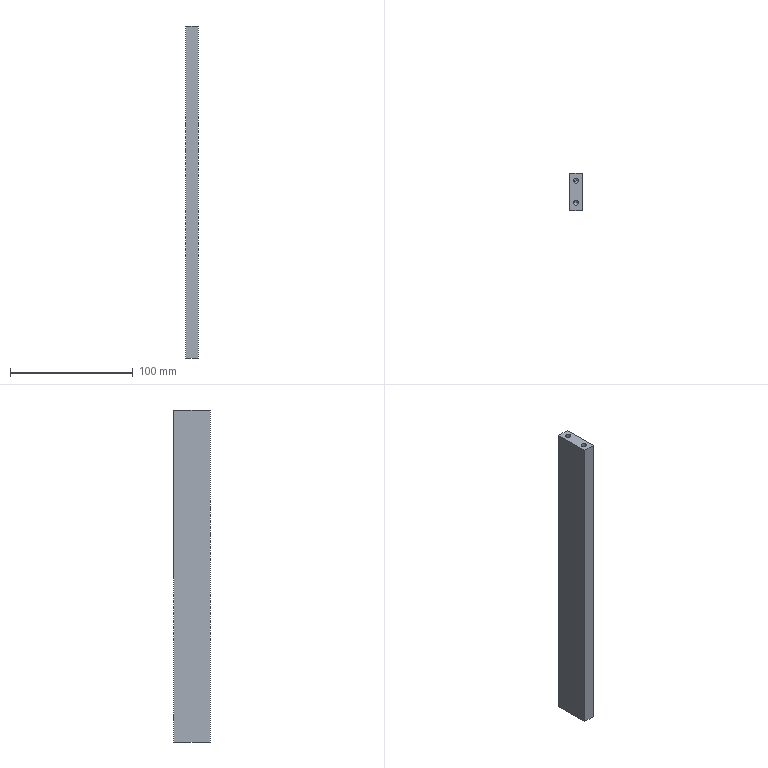Component | SolidWorks | LD101-02--Q1033-Q1-2-1 | 1 solid | 34 faces | box 10 x 30 x 270 mm | volume 79735 mm3 | cylinder 14 | cone 14 | plane 6 | commonest cylinder face diameters 4.2 x8 3.3 x6 | material AL6061
build123d program:
from build123d import *

# Parameters (mm, degrees)
SKETCH1_W                  = 270
SKETCH1_H                  = 30
BOSS_EXTRUDE1_DEPTH        = 5
M5_TAPPED_HOLE1_AT_2_COUNT = 2
M5_TAPPED_HOLE1_AT_2_PITCH = 18
M4_TAPPED_HOLE2_D          = 3.3
M4_TAPPED_HOLE2_DEPTH      = 13.5
M4_TAPPED_HOLE2_TIP        = 0.9914


with BuildPart() as part:
    # Sketch1 → Boss-Extrude1 (new, symmetric)
    with BuildSketch(Plane.XY):
        Rectangle(SKETCH1_W, SKETCH1_H)
    extrude(amount=BOSS_EXTRUDE1_DEPTH, both=True)

    # Sketch2 → M5 Tapped Hole1 (revolve, cut)
    with BuildSketch(Plane(origin=(135, -9, 0), x_dir=(0, 0, -1), z_dir=(0, 1, 0))):
        Polygon((0, 0), (0, 17.262), (2.1, 16), (2.1, 0), align=None)
    m5_tapped_hole1 = revolve(axis=Axis((141.35, -9, 0), (-1, 0, 0)), mode=Mode.SUBTRACT)

    # M5 Tapped Hole1 at 2: M5 Tapped Hole1 ×2
    with Locations(*[(0, i * M5_TAPPED_HOLE1_AT_2_PITCH, 0) for i in range(1, M5_TAPPED_HOLE1_AT_2_COUNT)]):
        add(m5_tapped_hole1, mode=Mode.SUBTRACT)

    # Mirror1: M5 Tapped Hole1 across plane
    add(m5_tapped_hole1.mirror(Plane(origin=(0, 0, 0), x_dir=(0, 0, 1), z_dir=(1, 0, 0))), mode=Mode.SUBTRACT)

    # Mirror1 copy 1 sketch → Mirror1 copy 1 (revolve, cut)
    with BuildSketch(Plane(origin=(-135, 9, 0), x_dir=(0, 0, -1), z_dir=(0, 1, 0))):
        Polygon((0, 0), (0, -17.262), (2.1, -16), (2.1, 0), align=None)
    revolve(axis=Axis((-141.35, 9, 0), (-1, 0, 0)), mode=Mode.SUBTRACT)

    # M4 Tapped Hole2
    with Locations(Plane(origin=(0, 15, 0), x_dir=(1, 0, 0), z_dir=(0, 1, 0))):
        with Locations((-115, 0), (115, 0), (0, 0)):
            Hole(M4_TAPPED_HOLE2_D / 2, depth=M4_TAPPED_HOLE2_DEPTH)
            with Locations((0, 0, -(M4_TAPPED_HOLE2_DEPTH + M4_TAPPED_HOLE2_TIP / 2))):  # 118° drill point
                Cone(0, M4_TAPPED_HOLE2_D / 2, M4_TAPPED_HOLE2_TIP, mode=Mode.SUBTRACT)


solid = part.part

# Placed as in the assembly
solid = solid.moved(Location((-345.29, -171.897, 146.257), (0, 90, 0)))
STEP:
#1=COLOUR_RGB('',0.7922,0.8196,0.9333);
#2=FILL_AREA_STYLE_COLOUR('',#1);
#3=FILL_AREA_STYLE('',(#2));
#4=SURFACE_STYLE_FILL_AREA(#3);
#5=SURFACE_SIDE_STYLE('',(#4));
#6=SURFACE_STYLE_USAGE(.BOTH.,#5);
#7=PRESENTATION_STYLE_ASSIGNMENT((#6));
#8=CARTESIAN_POINT('',(-13.529,-6.709,1.231));
#9=VERTEX_POINT('',#8);
#10=CARTESIAN_POINT('',(-13.659,-6.709,1.231));
#11=VERTEX_POINT('',#10);
#12=CARTESIAN_POINT('',(-13.594,-6.709,1.231));
#13=DIRECTION('',(0.,1.,0.));
#14=DIRECTION('',(-1.,0.,0.));
#15=AXIS2_PLACEMENT_3D('',#12,#13,#14);
#16=CIRCLE('',#15,0.06496);
#17=EDGE_CURVE('',#9,#11,#16,.T.);
#18=ORIENTED_EDGE('',*,*,#17,.F.);
#19=CARTESIAN_POINT('',(-13.529,-6.177,1.231));
#20=VERTEX_POINT('',#19);
#21=CARTESIAN_POINT('',(-13.529,-6.177,1.231));
#22=DIRECTION('',(0.,1.,0.));
#23=VECTOR('',#22,39.37);
#24=LINE('',#21,#23);
#25=EDGE_CURVE('',#9,#20,#24,.T.);
#26=ORIENTED_EDGE('',*,*,#25,.T.);
#27=CARTESIAN_POINT('',(-13.659,-6.177,1.231));
#28=VERTEX_POINT('',#27);
#29=CARTESIAN_POINT('',(-13.594,-6.177,1.231));
#30=DIRECTION('',(0.,1.,0.));
#31=DIRECTION('',(-1.,0.,0.));
#32=AXIS2_PLACEMENT_3D('',#29,#30,#31);
#33=CIRCLE('',#32,0.06496);
#34=EDGE_CURVE('',#20,#28,#33,.T.);
#35=ORIENTED_EDGE('',*,*,#34,.T.);
#36=CARTESIAN_POINT('',(-13.659,-6.177,1.231));
#37=DIRECTION('',(0.,1.,0.));
#38=VECTOR('',#37,39.37);
#39=LINE('',#36,#38);
#40=EDGE_CURVE('',#11,#28,#39,.T.);
#41=ORIENTED_EDGE('',*,*,#40,.F.);
#42=EDGE_LOOP('',(#18,#26,#35,#41));
#43=FACE_OUTER_BOUND('',#42,.T.);
#44=CARTESIAN_POINT('',(-13.594,-6.177,1.231));
#45=DIRECTION('',(0.,1.,0.));
#46=DIRECTION('',(-1.,0.,0.));
#47=AXIS2_PLACEMENT_3D('',#44,#45,#46);
#48=CYLINDRICAL_SURFACE('',#47,0.06496);
#49=ADVANCED_FACE('',(#43),#48,.F.);
#50=CARTESIAN_POINT('',(-13.594,-6.748,1.231));
#51=VERTEX_POINT('',#50);
#52=CARTESIAN_POINT('',(-13.659,-6.709,1.231));
#53=DIRECTION('',(-0.8572,0.515,0.));
#54=VECTOR('',#53,39.37);
#55=LINE('',#52,#54);
#56=EDGE_CURVE('',#51,#11,#55,.T.);
#57=ORIENTED_EDGE('',*,*,#56,.F.);
#58=CARTESIAN_POINT('',(-13.529,-6.709,1.231));
#59=DIRECTION('',(0.8572,0.515,0.));
#60=VECTOR('',#59,39.37);
#61=LINE('',#58,#60);
#62=EDGE_CURVE('',#51,#9,#61,.T.);
#63=ORIENTED_EDGE('',*,*,#62,.T.);
#64=ORIENTED_EDGE('',*,*,#17,.T.);
#65=EDGE_LOOP('',(#57,#63,#64));
#66=FACE_OUTER_BOUND('',#65,.T.);
#67=CARTESIAN_POINT('',(-13.594,-6.709,1.231));
#68=DIRECTION('',(0.,1.,0.));
#69=DIRECTION('',(-1.,0.,0.));
#70=AXIS2_PLACEMENT_3D('',#67,#68,#69);
#71=CONICAL_SURFACE('',#70,0.06496,1.03);
#72=ADVANCED_FACE('',(#66),#71,.F.);
#73=CARTESIAN_POINT('',(-13.529,-6.709,10.286));
#74=VERTEX_POINT('',#73);
#75=CARTESIAN_POINT('',(-13.659,-6.709,10.286));
#76=VERTEX_POINT('',#75);
#77=CARTESIAN_POINT('',(-13.594,-6.709,10.286));
#78=DIRECTION('',(0.,1.,0.));
#79=DIRECTION('',(-1.,0.,0.));
#80=AXIS2_PLACEMENT_3D('',#77,#78,#79);
#81=CIRCLE('',#80,0.06496);
#82=EDGE_CURVE('',#74,#76,#81,.T.);
#83=ORIENTED_EDGE('',*,*,#82,.F.);
#84=CARTESIAN_POINT('',(-13.529,-6.177,10.286));
#85=VERTEX_POINT('',#84);
#86=CARTESIAN_POINT('',(-13.529,-6.177,10.286));
#87=DIRECTION('',(0.,1.,0.));
#88=VECTOR('',#87,39.37);
#89=LINE('',#86,#88);
#90=EDGE_CURVE('',#74,#85,#89,.T.);
#91=ORIENTED_EDGE('',*,*,#90,.T.);
#92=CARTESIAN_POINT('',(-13.659,-6.177,10.286));
#93=VERTEX_POINT('',#92);
#94=CARTESIAN_POINT('',(-13.594,-6.177,10.286));
#95=DIRECTION('',(0.,1.,0.));
#96=DIRECTION('',(-1.,0.,0.));
#97=AXIS2_PLACEMENT_3D('',#94,#95,#96);
#98=CIRCLE('',#97,0.06496);
#99=EDGE_CURVE('',#85,#93,#98,.T.);
#100=ORIENTED_EDGE('',*,*,#99,.T.);
#101=CARTESIAN_POINT('',(-13.659,-6.177,10.286));
#102=DIRECTION('',(0.,1.,0.));
#103=VECTOR('',#102,39.37);
#104=LINE('',#101,#103);
#105=EDGE_CURVE('',#76,#93,#104,.T.);
#106=ORIENTED_EDGE('',*,*,#105,.F.);
#107=EDGE_LOOP('',(#83,#91,#100,#106));
#108=FACE_OUTER_BOUND('',#107,.T.);
#109=CARTESIAN_POINT('',(-13.594,-6.177,10.286));
#110=DIRECTION('',(0.,1.,0.));
#111=DIRECTION('',(-1.,0.,0.));
#112=AXIS2_PLACEMENT_3D('',#109,#110,#111);
#113=CYLINDRICAL_SURFACE('',#112,0.06496);
#114=ADVANCED_FACE('',(#108),#113,.F.);
#115=CARTESIAN_POINT('',(-13.594,-6.748,10.286));
#116=VERTEX_POINT('',#115);
#117=CARTESIAN_POINT('',(-13.659,-6.709,10.286));
#118=DIRECTION('',(-0.8572,0.515,0.));
#119=VECTOR('',#118,39.37);
#120=LINE('',#117,#119);
#121=EDGE_CURVE('',#116,#76,#120,.T.);
#122=ORIENTED_EDGE('',*,*,#121,.F.);
#123=CARTESIAN_POINT('',(-13.529,-6.709,10.286));
#124=DIRECTION('',(0.8572,0.515,0.));
#125=VECTOR('',#124,39.37);
#126=LINE('',#123,#125);
#127=EDGE_CURVE('',#116,#74,#126,.T.);
#128=ORIENTED_EDGE('',*,*,#127,.T.);
#129=ORIENTED_EDGE('',*,*,#82,.T.);
#130=EDGE_LOOP('',(#122,#128,#129));
#131=FACE_OUTER_BOUND('',#130,.T.);
#132=CARTESIAN_POINT('',(-13.594,-6.709,10.286));
#133=DIRECTION('',(0.,1.,0.));
#134=DIRECTION('',(-1.,0.,0.));
#135=AXIS2_PLACEMENT_3D('',#132,#133,#134);
#136=CONICAL_SURFACE('',#135,0.06496,1.03);
#137=ADVANCED_FACE('',(#131),#136,.F.);
#138=CARTESIAN_POINT('',(-13.529,-6.709,5.758));
#139=VERTEX_POINT('',#138);
#140=CARTESIAN_POINT('',(-13.659,-6.709,5.758));
#141=VERTEX_POINT('',#140);
#142=CARTESIAN_POINT('',(-13.594,-6.709,5.758));
#143=DIRECTION('',(0.,1.,0.));
#144=DIRECTION('',(-1.,0.,0.));
#145=AXIS2_PLACEMENT_3D('',#142,#143,#144);
#146=CIRCLE('',#145,0.06496);
#147=EDGE_CURVE('',#139,#141,#146,.T.);
#148=ORIENTED_EDGE('',*,*,#147,.F.);
#149=CARTESIAN_POINT('',(-13.529,-6.177,5.758));
#150=VERTEX_POINT('',#149);
#151=CARTESIAN_POINT('',(-13.529,-6.177,5.758));
#152=DIRECTION('',(0.,1.,0.));
#153=VECTOR('',#152,39.37);
#154=LINE('',#151,#153);
#155=EDGE_CURVE('',#139,#150,#154,.T.);
#156=ORIENTED_EDGE('',*,*,#155,.T.);
#157=CARTESIAN_POINT('',(-13.659,-6.177,5.758));
#158=VERTEX_POINT('',#157);
#159=CARTESIAN_POINT('',(-13.594,-6.177,5.758));
#160=DIRECTION('',(0.,1.,0.));
#161=DIRECTION('',(-1.,0.,0.));
#162=AXIS2_PLACEMENT_3D('',#159,#160,#161);
#163=CIRCLE('',#162,0.06496);
#164=EDGE_CURVE('',#150,#158,#163,.T.);
#165=ORIENTED_EDGE('',*,*,#164,.T.);
#166=CARTESIAN_POINT('',(-13.659,-6.177,5.758));
#167=DIRECTION('',(0.,1.,0.));
#168=VECTOR('',#167,39.37);
#169=LINE('',#166,#168);
#170=EDGE_CURVE('',#141,#158,#169,.T.);
#171=ORIENTED_EDGE('',*,*,#170,.F.);
#172=EDGE_LOOP('',(#148,#156,#165,#171));
#173=FACE_OUTER_BOUND('',#172,.T.);
#174=CARTESIAN_POINT('',(-13.594,-6.177,5.758));
#175=DIRECTION('',(0.,1.,0.));
#176=DIRECTION('',(-1.,0.,0.));
#177=AXIS2_PLACEMENT_3D('',#174,#175,#176);
#178=CYLINDRICAL_SURFACE('',#177,0.06496);
#179=ADVANCED_FACE('',(#173),#178,.F.);
#180=CARTESIAN_POINT('',(-13.594,-6.748,5.758));
#181=VERTEX_POINT('',#180);
#182=CARTESIAN_POINT('',(-13.659,-6.709,5.758));
#183=DIRECTION('',(-0.8572,0.515,0.));
#184=VECTOR('',#183,39.37);
#185=LINE('',#182,#184);
#186=EDGE_CURVE('',#181,#141,#185,.T.);
#187=ORIENTED_EDGE('',*,*,#186,.F.);
#188=CARTESIAN_POINT('',(-13.529,-6.709,5.758));
#189=DIRECTION('',(0.8572,0.515,0.));
#190=VECTOR('',#189,39.37);
#191=LINE('',#188,#190);
#192=EDGE_CURVE('',#181,#139,#191,.T.);
#193=ORIENTED_EDGE('',*,*,#192,.T.);
#194=ORIENTED_EDGE('',*,*,#147,.T.);
#195=EDGE_LOOP('',(#187,#193,#194));
#196=FACE_OUTER_BOUND('',#195,.T.);
#197=CARTESIAN_POINT('',(-13.594,-6.709,5.758));
#198=DIRECTION('',(0.,1.,0.));
#199=DIRECTION('',(-1.,0.,0.));
#200=AXIS2_PLACEMENT_3D('',#197,#198,#199);
#201=CONICAL_SURFACE('',#200,0.06496,1.03);
#202=ADVANCED_FACE('',(#196),#201,.F.);
#203=CARTESIAN_POINT('',(-13.511,-7.122,1.073));
#204=VERTEX_POINT('',#203);
#205=CARTESIAN_POINT('',(-13.677,-7.122,1.073));
#206=VERTEX_POINT('',#205);
#207=CARTESIAN_POINT('',(-13.594,-7.122,1.073));
#208=DIRECTION('',(-0.,0.,-1.));
#209=DIRECTION('',(-1.,0.,0.));
#210=AXIS2_PLACEMENT_3D('',#207,#208,#209);
#211=CIRCLE('',#210,0.08268);
#212=EDGE_CURVE('',#204,#206,#211,.T.);
#213=ORIENTED_EDGE('',*,*,#212,.F.);
#214=CARTESIAN_POINT('',(-13.511,-7.122,0.4432));
#215=VERTEX_POINT('',#214);
#216=CARTESIAN_POINT('',(-13.511,-7.122,0.4432));
#217=DIRECTION('',(-0.,0.,-1.));
#218=VECTOR('',#217,39.37);
#219=LINE('',#216,#218);
#220=EDGE_CURVE('',#204,#215,#219,.T.);
#221=ORIENTED_EDGE('',*,*,#220,.T.);
#222=CARTESIAN_POINT('',(-13.677,-7.122,0.4432));
#223=VERTEX_POINT('',#222);
#224=CARTESIAN_POINT('',(-13.594,-7.122,0.4432));
#225=DIRECTION('',(-0.,0.,-1.));
#226=DIRECTION('',(-1.,0.,0.));
#227=AXIS2_PLACEMENT_3D('',#224,#225,#226);
#228=CIRCLE('',#227,0.08268);
#229=EDGE_CURVE('',#215,#223,#228,.T.);
#230=ORIENTED_EDGE('',*,*,#229,.T.);
#231=CARTESIAN_POINT('',(-13.677,-7.122,0.4432));
#232=DIRECTION('',(-0.,0.,-1.));
#233=VECTOR('',#232,39.37);
#234=LINE('',#231,#233);
#235=EDGE_CURVE('',#206,#223,#234,.T.);
#236=ORIENTED_EDGE('',*,*,#235,.F.);
#237=EDGE_LOOP('',(#213,#221,#230,#236));
#238=FACE_OUTER_BOUND('',#237,.T.);
#239=CARTESIAN_POINT('',(-13.594,-7.122,0.4432));
#240=DIRECTION('',(-0.,0.,-1.));
#241=DIRECTION('',(-1.,0.,0.));
#242=AXIS2_PLACEMENT_3D('',#239,#240,#241);
#243=CYLINDRICAL_SURFACE('',#242,0.08268);
#244=ADVANCED_FACE('',(#238),#243,.F.);
#245=CARTESIAN_POINT('',(-13.594,-7.122,1.123));
#246=VERTEX_POINT('',#245);
#247=CARTESIAN_POINT('',(-13.677,-7.122,1.073));
#248=DIRECTION('',(-0.8572,0.,-0.515));
#249=VECTOR('',#248,39.37);
#250=LINE('',#247,#249);
#251=EDGE_CURVE('',#246,#206,#250,.T.);
#252=ORIENTED_EDGE('',*,*,#251,.F.);
#253=CARTESIAN_POINT('',(-13.511,-7.122,1.073));
#254=DIRECTION('',(0.8572,0.,-0.515));
#255=VECTOR('',#254,39.37);
#256=LINE('',#253,#255);
#257=EDGE_CURVE('',#246,#204,#256,.T.);
#258=ORIENTED_EDGE('',*,*,#257,.T.);
#259=ORIENTED_EDGE('',*,*,#212,.T.);
#260=EDGE_LOOP('',(#252,#258,#259));
#261=FACE_OUTER_BOUND('',#260,.T.);
#262=CARTESIAN_POINT('',(-13.594,-7.122,1.073));
#263=DIRECTION('',(-0.,0.,-1.));
#264=DIRECTION('',(-1.,0.,0.));
#265=AXIS2_PLACEMENT_3D('',#262,#263,#264);
#266=CONICAL_SURFACE('',#265,0.08268,1.03);
#267=ADVANCED_FACE('',(#261),#266,.F.);
#268=CARTESIAN_POINT('',(-13.511,-6.413,1.073));
#269=VERTEX_POINT('',#268);
#270=CARTESIAN_POINT('',(-13.677,-6.413,1.073));
#271=VERTEX_POINT('',#270);
#272=CARTESIAN_POINT('',(-13.594,-6.413,1.073));
#273=DIRECTION('',(-0.,0.,-1.));
#274=DIRECTION('',(-1.,0.,0.));
#275=AXIS2_PLACEMENT_3D('',#272,#273,#274);
#276=CIRCLE('',#275,0.08268);
#277=EDGE_CURVE('',#269,#271,#276,.T.);
#278=ORIENTED_EDGE('',*,*,#277,.F.);
#279=CARTESIAN_POINT('',(-13.511,-6.413,0.4432));
#280=VERTEX_POINT('',#279);
#281=CARTESIAN_POINT('',(-13.511,-6.413,0.4432));
#282=DIRECTION('',(-0.,0.,-1.));
#283=VECTOR('',#282,39.37);
#284=LINE('',#281,#283);
#285=EDGE_CURVE('',#269,#280,#284,.T.);
#286=ORIENTED_EDGE('',*,*,#285,.T.);
#287=CARTESIAN_POINT('',(-13.677,-6.413,0.4432));
#288=VERTEX_POINT('',#287);
#289=CARTESIAN_POINT('',(-13.594,-6.413,0.4432));
#290=DIRECTION('',(-0.,0.,-1.));
#291=DIRECTION('',(-1.,0.,0.));
#292=AXIS2_PLACEMENT_3D('',#289,#290,#291);
#293=CIRCLE('',#292,0.08268);
#294=EDGE_CURVE('',#280,#288,#293,.T.);
#295=ORIENTED_EDGE('',*,*,#294,.T.);
#296=CARTESIAN_POINT('',(-13.677,-6.413,0.4432));
#297=DIRECTION('',(-0.,0.,-1.));
#298=VECTOR('',#297,39.37);
#299=LINE('',#296,#298);
#300=EDGE_CURVE('',#271,#288,#299,.T.);
#301=ORIENTED_EDGE('',*,*,#300,.F.);
#302=EDGE_LOOP('',(#278,#286,#295,#301));
#303=FACE_OUTER_BOUND('',#302,.T.);
#304=CARTESIAN_POINT('',(-13.594,-6.413,0.4432));
#305=DIRECTION('',(-0.,0.,-1.));
#306=DIRECTION('',(-1.,0.,0.));
#307=AXIS2_PLACEMENT_3D('',#304,#305,#306);
#308=CYLINDRICAL_SURFACE('',#307,0.08268);
#309=ADVANCED_FACE('',(#303),#308,.F.);
#310=CARTESIAN_POINT('',(-13.594,-6.413,1.123));
#311=VERTEX_POINT('',#310);
#312=CARTESIAN_POINT('',(-13.677,-6.413,1.073));
#313=DIRECTION('',(-0.8572,0.,-0.515));
#314=VECTOR('',#313,39.37);
#315=LINE('',#312,#314);
#316=EDGE_CURVE('',#311,#271,#315,.T.);
#317=ORIENTED_EDGE('',*,*,#316,.F.);
#318=CARTESIAN_POINT('',(-13.511,-6.413,1.073));
#319=DIRECTION('',(0.8572,0.,-0.515));
#320=VECTOR('',#319,39.37);
#321=LINE('',#318,#320);
#322=EDGE_CURVE('',#311,#269,#321,.T.);
#323=ORIENTED_EDGE('',*,*,#322,.T.);
#324=ORIENTED_EDGE('',*,*,#277,.T.);
#325=EDGE_LOOP('',(#317,#323,#324));
#326=FACE_OUTER_BOUND('',#325,.T.);
#327=CARTESIAN_POINT('',(-13.594,-6.413,1.073));
#328=DIRECTION('',(-0.,0.,-1.));
#329=DIRECTION('',(-1.,0.,0.));
#330=AXIS2_PLACEMENT_3D('',#327,#328,#329);
#331=CONICAL_SURFACE('',#330,0.08268,1.03);
#332=ADVANCED_FACE('',(#326),#331,.F.);
#333=CARTESIAN_POINT('',(-13.677,-7.122,10.443));
#334=VERTEX_POINT('',#333);
#335=CARTESIAN_POINT('',(-13.511,-7.122,10.443));
#336=VERTEX_POINT('',#335);
#337=CARTESIAN_POINT('',(-13.594,-7.122,10.443));
#338=DIRECTION('',(0.,-0.,1.));
#339=DIRECTION('',(1.,0.,0.));
#340=AXIS2_PLACEMENT_3D('',#337,#338,#339);
#341=CIRCLE('',#340,0.08268);
#342=EDGE_CURVE('',#334,#336,#341,.T.);
#343=ORIENTED_EDGE('',*,*,#342,.F.);
#344=CARTESIAN_POINT('',(-13.677,-7.122,11.073));
#345=VERTEX_POINT('',#344);
#346=CARTESIAN_POINT('',(-13.677,-7.122,11.073));
#347=DIRECTION('',(0.,-0.,1.));
#348=VECTOR('',#347,39.37);
#349=LINE('',#346,#348);
#350=EDGE_CURVE('',#334,#345,#349,.T.);
#351=ORIENTED_EDGE('',*,*,#350,.T.);
#352=CARTESIAN_POINT('',(-13.511,-7.122,11.073));
#353=VERTEX_POINT('',#352);
#354=CARTESIAN_POINT('',(-13.594,-7.122,11.073));
#355=DIRECTION('',(0.,-0.,1.));
#356=DIRECTION('',(1.,0.,0.));
#357=AXIS2_PLACEMENT_3D('',#354,#355,#356);
#358=CIRCLE('',#357,0.08268);
#359=EDGE_CURVE('',#345,#353,#358,.T.);
#360=ORIENTED_EDGE('',*,*,#359,.T.);
#361=CARTESIAN_POINT('',(-13.511,-7.122,11.073));
#362=DIRECTION('',(0.,-0.,1.));
#363=VECTOR('',#362,39.37);
#364=LINE('',#361,#363);
#365=EDGE_CURVE('',#336,#353,#364,.T.);
#366=ORIENTED_EDGE('',*,*,#365,.F.);
#367=EDGE_LOOP('',(#343,#351,#360,#366));
#368=FACE_OUTER_BOUND('',#367,.T.);
#369=CARTESIAN_POINT('',(-13.594,-7.122,11.073));
#370=DIRECTION('',(0.,-0.,1.));
#371=DIRECTION('',(1.,0.,0.));
#372=AXIS2_PLACEMENT_3D('',#369,#370,#371);
#373=CYLINDRICAL_SURFACE('',#372,0.08268);
#374=ADVANCED_FACE('',(#368),#373,.F.);
#375=CARTESIAN_POINT('',(-13.594,-7.122,10.393));
#376=VERTEX_POINT('',#375);
#377=CARTESIAN_POINT('',(-13.511,-7.122,10.443));
#378=DIRECTION('',(0.8572,-0.,0.515));
#379=VECTOR('',#378,39.37);
#380=LINE('',#377,#379);
#381=EDGE_CURVE('',#376,#336,#380,.T.);
#382=ORIENTED_EDGE('',*,*,#381,.F.);
#383=CARTESIAN_POINT('',(-13.677,-7.122,10.443));
#384=DIRECTION('',(-0.8572,0.,0.515));
#385=VECTOR('',#384,39.37);
#386=LINE('',#383,#385);
#387=EDGE_CURVE('',#376,#334,#386,.T.);
#388=ORIENTED_EDGE('',*,*,#387,.T.);
#389=ORIENTED_EDGE('',*,*,#342,.T.);
#390=EDGE_LOOP('',(#382,#388,#389));
#391=FACE_OUTER_BOUND('',#390,.T.);
#392=CARTESIAN_POINT('',(-13.594,-7.122,10.443));
#393=DIRECTION('',(0.,-0.,1.));
#394=DIRECTION('',(1.,0.,0.));
#395=AXIS2_PLACEMENT_3D('',#392,#393,#394);
#396=CONICAL_SURFACE('',#395,0.08268,1.03);
#397=ADVANCED_FACE('',(#391),#396,.F.);
#398=CARTESIAN_POINT('',(-13.677,-6.413,10.443));
#399=VERTEX_POINT('',#398);
#400=CARTESIAN_POINT('',(-13.511,-6.413,10.443));
#401=VERTEX_POINT('',#400);
#402=CARTESIAN_POINT('',(-13.594,-6.413,10.443));
#403=DIRECTION('',(0.,-0.,1.));
#404=DIRECTION('',(1.,0.,0.));
#405=AXIS2_PLACEMENT_3D('',#402,#403,#404);
#406=CIRCLE('',#405,0.08268);
#407=EDGE_CURVE('',#399,#401,#406,.T.);
#408=ORIENTED_EDGE('',*,*,#407,.F.);
#409=CARTESIAN_POINT('',(-13.677,-6.413,11.073));
#410=VERTEX_POINT('',#409);
#411=CARTESIAN_POINT('',(-13.677,-6.413,11.073));
#412=DIRECTION('',(0.,-0.,1.));
#413=VECTOR('',#412,39.37);
#414=LINE('',#411,#413);
#415=EDGE_CURVE('',#399,#410,#414,.T.);
#416=ORIENTED_EDGE('',*,*,#415,.T.);
#417=CARTESIAN_POINT('',(-13.511,-6.413,11.073));
#418=VERTEX_POINT('',#417);
#419=CARTESIAN_POINT('',(-13.594,-6.413,11.073));
#420=DIRECTION('',(0.,-0.,1.));
#421=DIRECTION('',(1.,0.,0.));
#422=AXIS2_PLACEMENT_3D('',#419,#420,#421);
#423=CIRCLE('',#422,0.08268);
#424=EDGE_CURVE('',#410,#418,#423,.T.);
#425=ORIENTED_EDGE('',*,*,#424,.T.);
#426=CARTESIAN_POINT('',(-13.511,-6.413,11.073));
#427=DIRECTION('',(0.,-0.,1.));
#428=VECTOR('',#427,39.37);
#429=LINE('',#426,#428);
#430=EDGE_CURVE('',#401,#418,#429,.T.);
#431=ORIENTED_EDGE('',*,*,#430,.F.);
#432=EDGE_LOOP('',(#408,#416,#425,#431));
#433=FACE_OUTER_BOUND('',#432,.T.);
#434=CARTESIAN_POINT('',(-13.594,-6.413,11.073));
#435=DIRECTION('',(0.,-0.,1.));
#436=DIRECTION('',(1.,0.,0.));
#437=AXIS2_PLACEMENT_3D('',#434,#435,#436);
#438=CYLINDRICAL_SURFACE('',#437,0.08268);
#439=ADVANCED_FACE('',(#433),#438,.F.);
#440=CARTESIAN_POINT('',(-13.594,-6.413,10.393));
#441=VERTEX_POINT('',#440);
#442=CARTESIAN_POINT('',(-13.511,-6.413,10.443));
#443=DIRECTION('',(0.8572,-0.,0.515));
#444=VECTOR('',#443,39.37);
#445=LINE('',#442,#444);
#446=EDGE_CURVE('',#441,#401,#445,.T.);
#447=ORIENTED_EDGE('',*,*,#446,.F.);
#448=CARTESIAN_POINT('',(-13.677,-6.413,10.443));
#449=DIRECTION('',(-0.8572,0.,0.515));
#450=VECTOR('',#449,39.37);
#451=LINE('',#448,#450);
#452=EDGE_CURVE('',#441,#399,#451,.T.);
#453=ORIENTED_EDGE('',*,*,#452,.T.);
#454=ORIENTED_EDGE('',*,*,#407,.T.);
#455=EDGE_LOOP('',(#447,#453,#454));
#456=FACE_OUTER_BOUND('',#455,.T.);
#457=CARTESIAN_POINT('',(-13.594,-6.413,10.443));
#458=DIRECTION('',(0.,-0.,1.));
#459=DIRECTION('',(1.,0.,0.));
#460=AXIS2_PLACEMENT_3D('',#457,#458,#459);
#461=CONICAL_SURFACE('',#460,0.08268,1.03);
#462=ADVANCED_FACE('',(#456),#461,.F.);
#463=CARTESIAN_POINT('',(-13.594,-7.122,11.073));
#464=DIRECTION('',(0.,-0.,1.));
#465=DIRECTION('',(1.,0.,0.));
#466=AXIS2_PLACEMENT_3D('',#463,#464,#465);
#467=CIRCLE('',#466,0.08268);
#468=EDGE_CURVE('',#353,#345,#467,.T.);
#469=ORIENTED_EDGE('',*,*,#468,.F.);
#470=ORIENTED_EDGE('',*,*,#359,.F.);
#471=EDGE_LOOP('',(#469,#470));
#472=FACE_BOUND('',#471,.T.);
#473=CARTESIAN_POINT('',(-13.594,-6.413,11.073));
#474=DIRECTION('',(0.,-0.,1.));
#475=DIRECTION('',(1.,0.,0.));
#476=AXIS2_PLACEMENT_3D('',#473,#474,#475);
#477=CIRCLE('',#476,0.08268);
#478=EDGE_CURVE('',#418,#410,#477,.T.);
#479=ORIENTED_EDGE('',*,*,#478,.F.);
#480=ORIENTED_EDGE('',*,*,#424,.F.);
#481=EDGE_LOOP('',(#479,#480));
#482=FACE_BOUND('',#481,.T.);
#483=CARTESIAN_POINT('',(-13.397,-7.358,11.073));
#484=VERTEX_POINT('',#483);
#485=CARTESIAN_POINT('',(-13.397,-6.177,11.073));
#486=VERTEX_POINT('',#485);
#487=CARTESIAN_POINT('',(-13.397,-7.358,11.073));
#488=DIRECTION('',(0.,1.,0.));
#489=VECTOR('',#488,39.37);
#490=LINE('',#487,#489);
#491=EDGE_CURVE('',#484,#486,#490,.T.);
#492=ORIENTED_EDGE('',*,*,#491,.T.);
#493=CARTESIAN_POINT('',(-13.791,-6.177,11.073));
#494=VERTEX_POINT('',#493);
#495=CARTESIAN_POINT('',(-13.791,-6.177,11.073));
#496=DIRECTION('',(1.,0.,-0.));
#497=VECTOR('',#496,39.37);
#498=LINE('',#495,#497);
#499=EDGE_CURVE('',#494,#486,#498,.T.);
#500=ORIENTED_EDGE('',*,*,#499,.F.);
#501=CARTESIAN_POINT('',(-13.791,-7.358,11.073));
#502=VERTEX_POINT('',#501);
#503=CARTESIAN_POINT('',(-13.791,-7.358,11.073));
#504=DIRECTION('',(0.,1.,0.));
#505=VECTOR('',#504,39.37);
#506=LINE('',#503,#505);
#507=EDGE_CURVE('',#502,#494,#506,.T.);
#508=ORIENTED_EDGE('',*,*,#507,.F.);
#509=CARTESIAN_POINT('',(-13.791,-7.358,11.073));
#510=DIRECTION('',(1.,0.,-0.));
#511=VECTOR('',#510,39.37);
#512=LINE('',#509,#511);
#513=EDGE_CURVE('',#502,#484,#512,.T.);
#514=ORIENTED_EDGE('',*,*,#513,.T.);
#515=EDGE_LOOP('',(#492,#500,#508,#514));
#516=FACE_OUTER_BOUND('',#515,.T.);
#517=CARTESIAN_POINT('',(-13.791,-7.358,11.073));
#518=DIRECTION('',(-0.,0.,-1.));
#519=DIRECTION('',(-1.,-0.,0.));
#520=AXIS2_PLACEMENT_3D('',#517,#518,#519);
#521=PLANE('',#520);
#522=ADVANCED_FACE('',(#472,#482,#516),#521,.F.);
#523=CARTESIAN_POINT('',(-13.594,-6.177,1.231));
#524=DIRECTION('',(0.,1.,0.));
#525=DIRECTION('',(-1.,0.,0.));
#526=AXIS2_PLACEMENT_3D('',#523,#524,#525);
#527=CIRCLE('',#526,0.06496);
#528=EDGE_CURVE('',#28,#20,#527,.T.);
#529=ORIENTED_EDGE('',*,*,#528,.F.);
#530=ORIENTED_EDGE('',*,*,#34,.F.);
#531=EDGE_LOOP('',(#529,#530));
#532=FACE_BOUND('',#531,.T.);
#533=CARTESIAN_POINT('',(-13.594,-6.177,10.286));
#534=DIRECTION('',(0.,1.,0.));
#535=DIRECTION('',(-1.,0.,0.));
#536=AXIS2_PLACEMENT_3D('',#533,#534,#535);
#537=CIRCLE('',#536,0.06496);
#538=EDGE_CURVE('',#93,#85,#537,.T.);
#539=ORIENTED_EDGE('',*,*,#538,.F.);
#540=ORIENTED_EDGE('',*,*,#99,.F.);
#541=EDGE_LOOP('',(#539,#540));
#542=FACE_BOUND('',#541,.T.);
#543=CARTESIAN_POINT('',(-13.594,-6.177,5.758));
#544=DIRECTION('',(0.,1.,0.));
#545=DIRECTION('',(-1.,0.,0.));
#546=AXIS2_PLACEMENT_3D('',#543,#544,#545);
#547=CIRCLE('',#546,0.06496);
#548=EDGE_CURVE('',#158,#150,#547,.T.);
#549=ORIENTED_EDGE('',*,*,#548,.F.);
#550=ORIENTED_EDGE('',*,*,#164,.F.);
#551=EDGE_LOOP('',(#549,#550));
#552=FACE_BOUND('',#551,.T.);
#553=CARTESIAN_POINT('',(-13.397,-6.177,0.4432));
#554=VERTEX_POINT('',#553);
#555=CARTESIAN_POINT('',(-13.397,-6.177,0.4432));
#556=DIRECTION('',(-0.,0.,-1.));
#557=VECTOR('',#556,39.37);
#558=LINE('',#555,#557);
#559=EDGE_CURVE('',#486,#554,#558,.T.);
#560=ORIENTED_EDGE('',*,*,#559,.T.);
#561=CARTESIAN_POINT('',(-13.791,-6.177,0.4432));
#562=VERTEX_POINT('',#561);
#563=CARTESIAN_POINT('',(-13.791,-6.177,0.4432));
#564=DIRECTION('',(1.,0.,-0.));
#565=VECTOR('',#564,39.37);
#566=LINE('',#563,#565);
#567=EDGE_CURVE('',#562,#554,#566,.T.);
#568=ORIENTED_EDGE('',*,*,#567,.F.);
#569=CARTESIAN_POINT('',(-13.791,-6.177,0.4432));
#570=DIRECTION('',(-0.,0.,-1.));
#571=VECTOR('',#570,39.37);
#572=LINE('',#569,#571);
#573=EDGE_CURVE('',#494,#562,#572,.T.);
#574=ORIENTED_EDGE('',*,*,#573,.F.);
#575=ORIENTED_EDGE('',*,*,#499,.T.);
#576=EDGE_LOOP('',(#560,#568,#574,#575));
#577=FACE_OUTER_BOUND('',#576,.T.);
#578=CARTESIAN_POINT('',(-13.791,-6.177,0.4432));
#579=DIRECTION('',(0.,-1.,-0.));
#580=DIRECTION('',(1.,0.,-0.));
#581=AXIS2_PLACEMENT_3D('',#578,#579,#580);
#582=PLANE('',#581);
#583=ADVANCED_FACE('',(#532,#542,#552,#577),#582,.F.);
#584=CARTESIAN_POINT('',(-13.594,-7.122,0.4432));
#585=DIRECTION('',(-0.,0.,-1.));
#586=DIRECTION('',(-1.,0.,0.));
#587=AXIS2_PLACEMENT_3D('',#584,#585,#586);
#588=CIRCLE('',#587,0.08268);
#589=EDGE_CURVE('',#223,#215,#588,.T.);
#590=ORIENTED_EDGE('',*,*,#589,.F.);
#591=ORIENTED_EDGE('',*,*,#229,.F.);
#592=EDGE_LOOP('',(#590,#591));
#593=FACE_BOUND('',#592,.T.);
#594=CARTESIAN_POINT('',(-13.594,-6.413,0.4432));
#595=DIRECTION('',(-0.,0.,-1.));
#596=DIRECTION('',(-1.,0.,0.));
#597=AXIS2_PLACEMENT_3D('',#594,#595,#596);
#598=CIRCLE('',#597,0.08268);
#599=EDGE_CURVE('',#288,#280,#598,.T.);
#600=ORIENTED_EDGE('',*,*,#599,.F.);
#601=ORIENTED_EDGE('',*,*,#294,.F.);
#602=EDGE_LOOP('',(#600,#601));
#603=FACE_BOUND('',#602,.T.);
#604=CARTESIAN_POINT('',(-13.397,-7.358,0.4432));
#605=VERTEX_POINT('',#604);
#606=CARTESIAN_POINT('',(-13.397,-7.358,0.4432));
#607=DIRECTION('',(-0.,-1.,-0.));
#608=VECTOR('',#607,39.37);
#609=LINE('',#606,#608);
#610=EDGE_CURVE('',#554,#605,#609,.T.);
#611=ORIENTED_EDGE('',*,*,#610,.T.);
#612=CARTESIAN_POINT('',(-13.791,-7.358,0.4432));
#613=VERTEX_POINT('',#612);
#614=CARTESIAN_POINT('',(-13.791,-7.358,0.4432));
#615=DIRECTION('',(1.,0.,-0.));
#616=VECTOR('',#615,39.37);
#617=LINE('',#614,#616);
#618=EDGE_CURVE('',#613,#605,#617,.T.);
#619=ORIENTED_EDGE('',*,*,#618,.F.);
#620=CARTESIAN_POINT('',(-13.791,-7.358,0.4432));
#621=DIRECTION('',(-0.,-1.,-0.));
#622=VECTOR('',#621,39.37);
#623=LINE('',#620,#622);
#624=EDGE_CURVE('',#562,#613,#623,.T.);
#625=ORIENTED_EDGE('',*,*,#624,.F.);
#626=ORIENTED_EDGE('',*,*,#567,.T.);
#627=EDGE_LOOP('',(#611,#619,#625,#626));
#628=FACE_OUTER_BOUND('',#627,.T.);
#629=CARTESIAN_POINT('',(-13.791,-7.358,0.4432));
#630=DIRECTION('',(0.,-0.,1.));
#631=DIRECTION('',(1.,0.,-0.));
#632=AXIS2_PLACEMENT_3D('',#629,#630,#631);
#633=PLANE('',#632);
#634=ADVANCED_FACE('',(#593,#603,#628),#633,.F.);
#635=CARTESIAN_POINT('',(-13.397,-7.358,0.4432));
#636=DIRECTION('',(0.,-0.,1.));
#637=VECTOR('',#636,39.37);
#638=LINE('',#635,#637);
#639=EDGE_CURVE('',#605,#484,#638,.T.);
#640=ORIENTED_EDGE('',*,*,#639,.T.);
#641=ORIENTED_EDGE('',*,*,#513,.F.);
#642=CARTESIAN_POINT('',(-13.791,-7.358,0.4432));
#643=DIRECTION('',(0.,-0.,1.));
#644=VECTOR('',#643,39.37);
#645=LINE('',#642,#644);
#646=EDGE_CURVE('',#613,#502,#645,.T.);
#647=ORIENTED_EDGE('',*,*,#646,.F.);
#648=ORIENTED_EDGE('',*,*,#618,.T.);
#649=EDGE_LOOP('',(#640,#641,#647,#648));
#650=FACE_OUTER_BOUND('',#649,.T.);
#651=CARTESIAN_POINT('',(-13.791,-7.358,0.4432));
#652=DIRECTION('',(-0.,1.,0.));
#653=DIRECTION('',(-1.,-0.,0.));
#654=AXIS2_PLACEMENT_3D('',#651,#652,#653);
#655=PLANE('',#654);
#656=ADVANCED_FACE('',(#650),#655,.F.);
#657=ORIENTED_EDGE('',*,*,#507,.T.);
#658=ORIENTED_EDGE('',*,*,#573,.T.);
#659=ORIENTED_EDGE('',*,*,#624,.T.);
#660=ORIENTED_EDGE('',*,*,#646,.T.);
#661=EDGE_LOOP('',(#657,#658,#659,#660));
#662=FACE_OUTER_BOUND('',#661,.T.);
#663=CARTESIAN_POINT('',(-13.791,-6.768,5.758));
#664=DIRECTION('',(1.,0.,-0.));
#665=DIRECTION('',(-0.,0.,-1.));
#666=AXIS2_PLACEMENT_3D('',#663,#664,#665);
#667=PLANE('',#666);
#668=ADVANCED_FACE('',(#662),#667,.F.);
#669=ORIENTED_EDGE('',*,*,#491,.F.);
#670=ORIENTED_EDGE('',*,*,#639,.F.);
#671=ORIENTED_EDGE('',*,*,#610,.F.);
#672=ORIENTED_EDGE('',*,*,#559,.F.);
#673=EDGE_LOOP('',(#669,#670,#671,#672));
#674=FACE_OUTER_BOUND('',#673,.T.);
#675=CARTESIAN_POINT('',(-13.397,-6.768,5.758));
#676=DIRECTION('',(1.,0.,-0.));
#677=DIRECTION('',(-0.,0.,-1.));
#678=AXIS2_PLACEMENT_3D('',#675,#676,#677);
#679=PLANE('',#678);
#680=ADVANCED_FACE('',(#674),#679,.T.);
#681=ORIENTED_EDGE('',*,*,#452,.F.);
#682=ORIENTED_EDGE('',*,*,#446,.T.);
#683=CARTESIAN_POINT('',(-13.594,-6.413,10.443));
#684=DIRECTION('',(0.,-0.,1.));
#685=DIRECTION('',(1.,0.,0.));
#686=AXIS2_PLACEMENT_3D('',#683,#684,#685);
#687=CIRCLE('',#686,0.08268);
#688=EDGE_CURVE('',#401,#399,#687,.T.);
#689=ORIENTED_EDGE('',*,*,#688,.T.);
#690=EDGE_LOOP('',(#681,#682,#689));
#691=FACE_OUTER_BOUND('',#690,.T.);
#692=CARTESIAN_POINT('',(-13.594,-6.413,10.443));
#693=DIRECTION('',(0.,-0.,1.));
#694=DIRECTION('',(1.,0.,0.));
#695=AXIS2_PLACEMENT_3D('',#692,#693,#694);
#696=CONICAL_SURFACE('',#695,0.08268,1.03);
#697=ADVANCED_FACE('',(#691),#696,.F.);
#698=ORIENTED_EDGE('',*,*,#415,.F.);
#699=ORIENTED_EDGE('',*,*,#688,.F.);
#700=ORIENTED_EDGE('',*,*,#430,.T.);
#701=ORIENTED_EDGE('',*,*,#478,.T.);
#702=EDGE_LOOP('',(#698,#699,#700,#701));
#703=FACE_OUTER_BOUND('',#702,.T.);
#704=CARTESIAN_POINT('',(-13.594,-6.413,11.073));
#705=DIRECTION('',(0.,-0.,1.));
#706=DIRECTION('',(1.,0.,0.));
#707=AXIS2_PLACEMENT_3D('',#704,#705,#706);
#708=CYLINDRICAL_SURFACE('',#707,0.08268);
#709=ADVANCED_FACE('',(#703),#708,.F.);
#710=ORIENTED_EDGE('',*,*,#387,.F.);
#711=ORIENTED_EDGE('',*,*,#381,.T.);
#712=CARTESIAN_POINT('',(-13.594,-7.122,10.443));
#713=DIRECTION('',(0.,-0.,1.));
#714=DIRECTION('',(1.,0.,0.));
#715=AXIS2_PLACEMENT_3D('',#712,#713,#714);
#716=CIRCLE('',#715,0.08268);
#717=EDGE_CURVE('',#336,#334,#716,.T.);
#718=ORIENTED_EDGE('',*,*,#717,.T.);
#719=EDGE_LOOP('',(#710,#711,#718));
#720=FACE_OUTER_BOUND('',#719,.T.);
#721=CARTESIAN_POINT('',(-13.594,-7.122,10.443));
#722=DIRECTION('',(0.,-0.,1.));
#723=DIRECTION('',(1.,0.,0.));
#724=AXIS2_PLACEMENT_3D('',#721,#722,#723);
#725=CONICAL_SURFACE('',#724,0.08268,1.03);
#726=ADVANCED_FACE('',(#720),#725,.F.);
#727=ORIENTED_EDGE('',*,*,#350,.F.);
#728=ORIENTED_EDGE('',*,*,#717,.F.);
#729=ORIENTED_EDGE('',*,*,#365,.T.);
#730=ORIENTED_EDGE('',*,*,#468,.T.);
#731=EDGE_LOOP('',(#727,#728,#729,#730));
#732=FACE_OUTER_BOUND('',#731,.T.);
#733=CARTESIAN_POINT('',(-13.594,-7.122,11.073));
#734=DIRECTION('',(0.,-0.,1.));
#735=DIRECTION('',(1.,0.,0.));
#736=AXIS2_PLACEMENT_3D('',#733,#734,#735);
#737=CYLINDRICAL_SURFACE('',#736,0.08268);
#738=ADVANCED_FACE('',(#732),#737,.F.);
#739=ORIENTED_EDGE('',*,*,#322,.F.);
#740=ORIENTED_EDGE('',*,*,#316,.T.);
#741=CARTESIAN_POINT('',(-13.594,-6.413,1.073));
#742=DIRECTION('',(-0.,0.,-1.));
#743=DIRECTION('',(-1.,0.,0.));
#744=AXIS2_PLACEMENT_3D('',#741,#742,#743);
#745=CIRCLE('',#744,0.08268);
#746=EDGE_CURVE('',#271,#269,#745,.T.);
#747=ORIENTED_EDGE('',*,*,#746,.T.);
#748=EDGE_LOOP('',(#739,#740,#747));
#749=FACE_OUTER_BOUND('',#748,.T.);
#750=CARTESIAN_POINT('',(-13.594,-6.413,1.073));
#751=DIRECTION('',(-0.,0.,-1.));
#752=DIRECTION('',(-1.,0.,0.));
#753=AXIS2_PLACEMENT_3D('',#750,#751,#752);
#754=CONICAL_SURFACE('',#753,0.08268,1.03);
#755=ADVANCED_FACE('',(#749),#754,.F.);
#756=ORIENTED_EDGE('',*,*,#285,.F.);
#757=ORIENTED_EDGE('',*,*,#746,.F.);
#758=ORIENTED_EDGE('',*,*,#300,.T.);
#759=ORIENTED_EDGE('',*,*,#599,.T.);
#760=EDGE_LOOP('',(#756,#757,#758,#759));
#761=FACE_OUTER_BOUND('',#760,.T.);
#762=CARTESIAN_POINT('',(-13.594,-6.413,0.4432));
#763=DIRECTION('',(-0.,0.,-1.));
#764=DIRECTION('',(-1.,0.,0.));
#765=AXIS2_PLACEMENT_3D('',#762,#763,#764);
#766=CYLINDRICAL_SURFACE('',#765,0.08268);
#767=ADVANCED_FACE('',(#761),#766,.F.);
#768=ORIENTED_EDGE('',*,*,#257,.F.);
#769=ORIENTED_EDGE('',*,*,#251,.T.);
#770=CARTESIAN_POINT('',(-13.594,-7.122,1.073));
#771=DIRECTION('',(-0.,0.,-1.));
#772=DIRECTION('',(-1.,0.,0.));
#773=AXIS2_PLACEMENT_3D('',#770,#771,#772);
#774=CIRCLE('',#773,0.08268);
#775=EDGE_CURVE('',#206,#204,#774,.T.);
#776=ORIENTED_EDGE('',*,*,#775,.T.);
#777=EDGE_LOOP('',(#768,#769,#776));
#778=FACE_OUTER_BOUND('',#777,.T.);
#779=CARTESIAN_POINT('',(-13.594,-7.122,1.073));
#780=DIRECTION('',(-0.,0.,-1.));
#781=DIRECTION('',(-1.,0.,0.));
#782=AXIS2_PLACEMENT_3D('',#779,#780,#781);
#783=CONICAL_SURFACE('',#782,0.08268,1.03);
#784=ADVANCED_FACE('',(#778),#783,.F.);
#785=ORIENTED_EDGE('',*,*,#220,.F.);
#786=ORIENTED_EDGE('',*,*,#775,.F.);
#787=ORIENTED_EDGE('',*,*,#235,.T.);
#788=ORIENTED_EDGE('',*,*,#589,.T.);
#789=EDGE_LOOP('',(#785,#786,#787,#788));
#790=FACE_OUTER_BOUND('',#789,.T.);
#791=CARTESIAN_POINT('',(-13.594,-7.122,0.4432));
#792=DIRECTION('',(-0.,0.,-1.));
#793=DIRECTION('',(-1.,0.,0.));
#794=AXIS2_PLACEMENT_3D('',#791,#792,#793);
#795=CYLINDRICAL_SURFACE('',#794,0.08268);
#796=ADVANCED_FACE('',(#790),#795,.F.);
#797=ORIENTED_EDGE('',*,*,#192,.F.);
#798=ORIENTED_EDGE('',*,*,#186,.T.);
#799=CARTESIAN_POINT('',(-13.594,-6.709,5.758));
#800=DIRECTION('',(0.,1.,0.));
#801=DIRECTION('',(-1.,0.,0.));
#802=AXIS2_PLACEMENT_3D('',#799,#800,#801);
#803=CIRCLE('',#802,0.06496);
#804=EDGE_CURVE('',#141,#139,#803,.T.);
#805=ORIENTED_EDGE('',*,*,#804,.T.);
#806=EDGE_LOOP('',(#797,#798,#805));
#807=FACE_OUTER_BOUND('',#806,.T.);
#808=CARTESIAN_POINT('',(-13.594,-6.709,5.758));
#809=DIRECTION('',(0.,1.,0.));
#810=DIRECTION('',(-1.,0.,0.));
#811=AXIS2_PLACEMENT_3D('',#808,#809,#810);
#812=CONICAL_SURFACE('',#811,0.06496,1.03);
#813=ADVANCED_FACE('',(#807),#812,.F.);
#814=ORIENTED_EDGE('',*,*,#155,.F.);
#815=ORIENTED_EDGE('',*,*,#804,.F.);
#816=ORIENTED_EDGE('',*,*,#170,.T.);
#817=ORIENTED_EDGE('',*,*,#548,.T.);
#818=EDGE_LOOP('',(#814,#815,#816,#817));
#819=FACE_OUTER_BOUND('',#818,.T.);
#820=CARTESIAN_POINT('',(-13.594,-6.177,5.758));
#821=DIRECTION('',(0.,1.,0.));
#822=DIRECTION('',(-1.,0.,0.));
#823=AXIS2_PLACEMENT_3D('',#820,#821,#822);
#824=CYLINDRICAL_SURFACE('',#823,0.06496);
#825=ADVANCED_FACE('',(#819),#824,.F.);
#826=ORIENTED_EDGE('',*,*,#127,.F.);
#827=ORIENTED_EDGE('',*,*,#121,.T.);
#828=CARTESIAN_POINT('',(-13.594,-6.709,10.286));
#829=DIRECTION('',(0.,1.,0.));
#830=DIRECTION('',(-1.,0.,0.));
#831=AXIS2_PLACEMENT_3D('',#828,#829,#830);
#832=CIRCLE('',#831,0.06496);
#833=EDGE_CURVE('',#76,#74,#832,.T.);
#834=ORIENTED_EDGE('',*,*,#833,.T.);
#835=EDGE_LOOP('',(#826,#827,#834));
#836=FACE_OUTER_BOUND('',#835,.T.);
#837=CARTESIAN_POINT('',(-13.594,-6.709,10.286));
#838=DIRECTION('',(0.,1.,0.));
#839=DIRECTION('',(-1.,0.,0.));
#840=AXIS2_PLACEMENT_3D('',#837,#838,#839);
#841=CONICAL_SURFACE('',#840,0.06496,1.03);
#842=ADVANCED_FACE('',(#836),#841,.F.);
#843=ORIENTED_EDGE('',*,*,#90,.F.);
#844=ORIENTED_EDGE('',*,*,#833,.F.);
#845=ORIENTED_EDGE('',*,*,#105,.T.);
#846=ORIENTED_EDGE('',*,*,#538,.T.);
#847=EDGE_LOOP('',(#843,#844,#845,#846));
#848=FACE_OUTER_BOUND('',#847,.T.);
#849=CARTESIAN_POINT('',(-13.594,-6.177,10.286));
#850=DIRECTION('',(0.,1.,0.));
#851=DIRECTION('',(-1.,0.,0.));
#852=AXIS2_PLACEMENT_3D('',#849,#850,#851);
#853=CYLINDRICAL_SURFACE('',#852,0.06496);
#854=ADVANCED_FACE('',(#848),#853,.F.);
#855=ORIENTED_EDGE('',*,*,#62,.F.);
#856=ORIENTED_EDGE('',*,*,#56,.T.);
#857=CARTESIAN_POINT('',(-13.594,-6.709,1.231));
#858=DIRECTION('',(0.,1.,0.));
#859=DIRECTION('',(-1.,0.,0.));
#860=AXIS2_PLACEMENT_3D('',#857,#858,#859);
#861=CIRCLE('',#860,0.06496);
#862=EDGE_CURVE('',#11,#9,#861,.T.);
#863=ORIENTED_EDGE('',*,*,#862,.T.);
#864=EDGE_LOOP('',(#855,#856,#863));
#865=FACE_OUTER_BOUND('',#864,.T.);
#866=CARTESIAN_POINT('',(-13.594,-6.709,1.231));
#867=DIRECTION('',(0.,1.,0.));
#868=DIRECTION('',(-1.,0.,0.));
#869=AXIS2_PLACEMENT_3D('',#866,#867,#868);
#870=CONICAL_SURFACE('',#869,0.06496,1.03);
#871=ADVANCED_FACE('',(#865),#870,.F.);
#872=ORIENTED_EDGE('',*,*,#25,.F.);
#873=ORIENTED_EDGE('',*,*,#862,.F.);
#874=ORIENTED_EDGE('',*,*,#40,.T.);
#875=ORIENTED_EDGE('',*,*,#528,.T.);
#876=EDGE_LOOP('',(#872,#873,#874,#875));
#877=FACE_OUTER_BOUND('',#876,.T.);
#878=CARTESIAN_POINT('',(-13.594,-6.177,1.231));
#879=DIRECTION('',(0.,1.,0.));
#880=DIRECTION('',(-1.,0.,0.));
#881=AXIS2_PLACEMENT_3D('',#878,#879,#880);
#882=CYLINDRICAL_SURFACE('',#881,0.06496);
#883=ADVANCED_FACE('',(#877),#882,.F.);
#884=CLOSED_SHELL('',(#49,#72,#114,#137,#179,#202,#244,#267,#309,#332,#374,#397,#439,#462,#522,#583,#634,#656,#668,#680,#697,#709,#726,#738,#755,#767,#784,#796,#813,#825,#842,#854,#871,#883));
#885=MANIFOLD_SOLID_BREP('',#884);
#886=STYLED_ITEM('',(#7),#885);
#887=(LENGTH_UNIT()NAMED_UNIT(*)SI_UNIT($,.METRE.));
#888=LENGTH_MEASURE_WITH_UNIT(LENGTH_MEASURE(0.0254),#887);
#889=DIMENSIONAL_EXPONENTS(1.,0.,0.,0.,0.,0.,0.);
#890=(CONVERSION_BASED_UNIT('',#888)LENGTH_UNIT()NAMED_UNIT(#889));
#891=UNCERTAINTY_MEASURE_WITH_UNIT(LENGTH_MEASURE(0.00001),#890,'','');
#892=(NAMED_UNIT(*)PLANE_ANGLE_UNIT()SI_UNIT($,.RADIAN.));
#893=(NAMED_UNIT(*)SI_UNIT($,.STERADIAN.)SOLID_ANGLE_UNIT());
#894=(GEOMETRIC_REPRESENTATION_CONTEXT(3)GLOBAL_UNCERTAINTY_ASSIGNED_CONTEXT((#891))GLOBAL_UNIT_ASSIGNED_CONTEXT((#890,#892,#893))REPRESENTATION_CONTEXT('',''));
#895=MECHANICAL_DESIGN_GEOMETRIC_PRESENTATION_REPRESENTATION('',(#886),#894);
#896=CARTESIAN_POINT('',(0.,0.,0.));
#897=DIRECTION('',(0.,0.,1.));
#898=DIRECTION('',(1.,0.,0.));
#899=AXIS2_PLACEMENT_3D('',#896,#897,#898);
#900=(LENGTH_UNIT()NAMED_UNIT(*)SI_UNIT($,.METRE.));
#901=LENGTH_MEASURE_WITH_UNIT(LENGTH_MEASURE(0.0254),#900);
#902=DIMENSIONAL_EXPONENTS(1.,0.,0.,0.,0.,0.,0.);
#903=(CONVERSION_BASED_UNIT('',#901)LENGTH_UNIT()NAMED_UNIT(#902));
#904=UNCERTAINTY_MEASURE_WITH_UNIT(LENGTH_MEASURE(0.00001),#903,'','');
#905=(NAMED_UNIT(*)PLANE_ANGLE_UNIT()SI_UNIT($,.RADIAN.));
#906=(NAMED_UNIT(*)SI_UNIT($,.STERADIAN.)SOLID_ANGLE_UNIT());
#907=(GEOMETRIC_REPRESENTATION_CONTEXT(3)GLOBAL_UNCERTAINTY_ASSIGNED_CONTEXT((#904))GLOBAL_UNIT_ASSIGNED_CONTEXT((#903,#905,#906))REPRESENTATION_CONTEXT('',''));
#908=ADVANCED_BREP_SHAPE_REPRESENTATION('',(#885,#899),#907);
#909=PRESENTATION_LAYER_ASSIGNMENT('','',(#886));